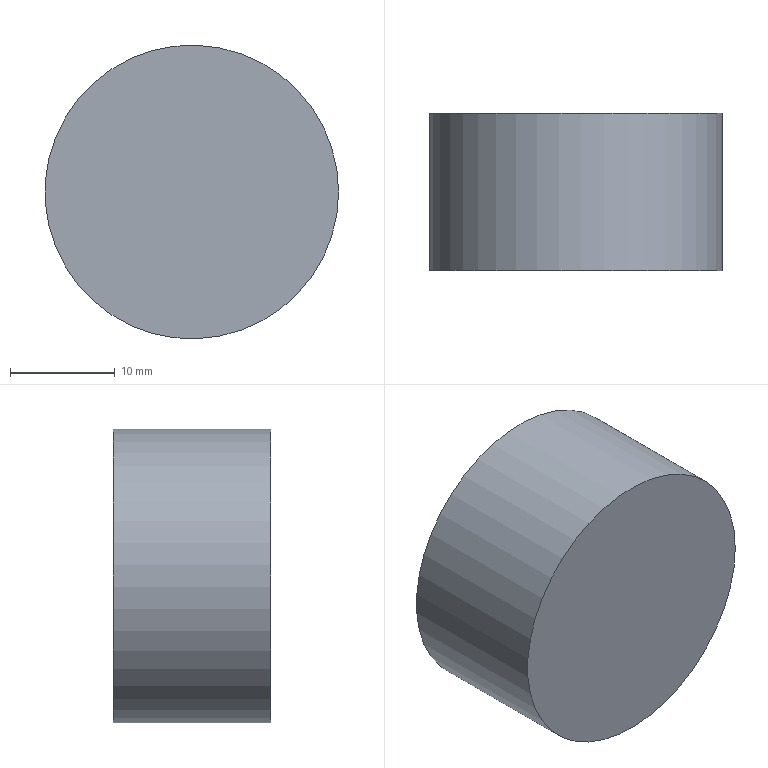Component | NX | CUP | 1 solid | 5 faces | box 28 x 15 x 28 mm | volume 5435 mm3 | plane 3 | cylinder 2 | commonest cylinder face diameters 28 x1 22 x1
STEP:
#1=CARTESIAN_POINT('',(0.,0.,0.));
#2=DIRECTION('',(0.,0.,1.));
#3=DIRECTION('',(1.,0.,0.));
#4=AXIS2_PLACEMENT_3D('',#1,#2,#3);
#5=CARTESIAN_POINT('',(14.,-47.923,-93.));
#6=VERTEX_POINT('',#5);
#7=CARTESIAN_POINT('',(0.,-47.923,-93.));
#8=DIRECTION('',(0.,1.,0.));
#9=DIRECTION('',(1.,0.,0.));
#10=AXIS2_PLACEMENT_3D('',#7,#8,#9);
#11=CIRCLE('',#10,14.);
#12=CARTESIAN_POINT('',(0.,-47.923,-93.));
#13=DIRECTION('',(0.,-1.,0.));
#14=DIRECTION('',(-1.,0.,0.));
#15=AXIS2_PLACEMENT_3D('',#12,#13,#14);
#16=CYLINDRICAL_SURFACE('',#15,14.);
#17=CARTESIAN_POINT('',(9.425,0.));
#18=DIRECTION('',(-1.,0.));
#19=VECTOR('',#18,1.);
#20=LINE('',#17,#19);
#21=(GEOMETRIC_REPRESENTATION_CONTEXT(2)PARAMETRIC_REPRESENTATION_CONTEXT()REPRESENTATION_CONTEXT('',''));
#22=DEFINITIONAL_REPRESENTATION('',(#20),#21);
#23=PCURVE('',#16,#22);
#24=CARTESIAN_POINT('',(0.,-47.923,-93.));
#25=DIRECTION('',(0.,1.,0.));
#26=DIRECTION('',(1.,0.,0.));
#27=AXIS2_PLACEMENT_3D('',#24,#25,#26);
#28=PLANE('',#27);
#29=CARTESIAN_POINT('',(0.,0.));
#30=DIRECTION('',(1.,0.));
#31=AXIS2_PLACEMENT_2D('',#29,#30);
#32=CIRCLE('',#31,14.);
#33=(GEOMETRIC_REPRESENTATION_CONTEXT(2)PARAMETRIC_REPRESENTATION_CONTEXT()REPRESENTATION_CONTEXT('',''));
#34=DEFINITIONAL_REPRESENTATION('',(#32),#33);
#35=PCURVE('',#28,#34);
#36=SURFACE_CURVE('',#11,(#23,#35),.PCURVE_S1.);
#37=EDGE_CURVE('',#6,#6,#36,.T.);
#38=ORIENTED_EDGE('',*,*,#37,.F.);
#39=CARTESIAN_POINT('',(14.,-62.923,-93.));
#40=VERTEX_POINT('',#39);
#41=CARTESIAN_POINT('',(14.,-47.923,-93.));
#42=CARTESIAN_POINT('',(14.,-62.923,-93.));
#43=B_SPLINE_CURVE_WITH_KNOTS('',1,(#41,#42),.UNSPECIFIED.,.F.,.F.,(2,2),(0.,15.),.PIECEWISE_BEZIER_KNOTS.);
#44=CARTESIAN_POINT('',(9.425,0.));
#45=DIRECTION('',(0.,1.));
#46=VECTOR('',#45,1.);
#47=LINE('',#44,#46);
#48=(GEOMETRIC_REPRESENTATION_CONTEXT(2)PARAMETRIC_REPRESENTATION_CONTEXT()REPRESENTATION_CONTEXT('',''));
#49=DEFINITIONAL_REPRESENTATION('',(#47),#48);
#50=PCURVE('',#16,#49);
#51=CARTESIAN_POINT('',(3.142,0.));
#52=DIRECTION('',(0.,1.));
#53=VECTOR('',#52,1.);
#54=LINE('',#51,#53);
#55=(GEOMETRIC_REPRESENTATION_CONTEXT(2)PARAMETRIC_REPRESENTATION_CONTEXT()REPRESENTATION_CONTEXT('',''));
#56=DEFINITIONAL_REPRESENTATION('',(#54),#55);
#57=PCURVE('',#16,#56);
#58=SEAM_CURVE('',#43,(#50,#57),.PCURVE_S1.);
#59=EDGE_CURVE('',#6,#40,#58,.T.);
#60=ORIENTED_EDGE('',*,*,#59,.T.);
#61=CARTESIAN_POINT('',(0.,-62.923,-93.));
#62=DIRECTION('',(0.,1.,0.));
#63=DIRECTION('',(1.,0.,0.));
#64=AXIS2_PLACEMENT_3D('',#61,#62,#63);
#65=CIRCLE('',#64,14.);
#66=CARTESIAN_POINT('',(9.425,15.));
#67=DIRECTION('',(-1.,0.));
#68=VECTOR('',#67,1.);
#69=LINE('',#66,#68);
#70=(GEOMETRIC_REPRESENTATION_CONTEXT(2)PARAMETRIC_REPRESENTATION_CONTEXT()REPRESENTATION_CONTEXT('',''));
#71=DEFINITIONAL_REPRESENTATION('',(#69),#70);
#72=PCURVE('',#16,#71);
#73=CARTESIAN_POINT('',(0.,-62.923,-93.));
#74=DIRECTION('',(0.,1.,0.));
#75=DIRECTION('',(1.,0.,0.));
#76=AXIS2_PLACEMENT_3D('',#73,#74,#75);
#77=PLANE('',#76);
#78=CARTESIAN_POINT('',(0.,0.));
#79=DIRECTION('',(1.,0.));
#80=AXIS2_PLACEMENT_2D('',#78,#79);
#81=CIRCLE('',#80,14.);
#82=(GEOMETRIC_REPRESENTATION_CONTEXT(2)PARAMETRIC_REPRESENTATION_CONTEXT()REPRESENTATION_CONTEXT('',''));
#83=DEFINITIONAL_REPRESENTATION('',(#81),#82);
#84=PCURVE('',#77,#83);
#85=SURFACE_CURVE('',#65,(#72,#84),.PCURVE_S1.);
#86=EDGE_CURVE('',#40,#40,#85,.T.);
#87=ORIENTED_EDGE('',*,*,#86,.T.);
#88=ORIENTED_EDGE('',*,*,#59,.F.);
#89=EDGE_LOOP('',(#38,#60,#87,#88));
#90=FACE_BOUND('',#89,.T.);
#91=ADVANCED_FACE('',(#90),#16,.T.);
#92=CARTESIAN_POINT('',(11.,-47.923,-93.));
#93=VERTEX_POINT('',#92);
#94=CARTESIAN_POINT('',(0.,-47.923,-93.));
#95=DIRECTION('',(0.,1.,0.));
#96=DIRECTION('',(1.,0.,0.));
#97=AXIS2_PLACEMENT_3D('',#94,#95,#96);
#98=CIRCLE('',#97,11.);
#99=CARTESIAN_POINT('',(0.,0.));
#100=DIRECTION('',(1.,0.));
#101=AXIS2_PLACEMENT_2D('',#99,#100);
#102=CIRCLE('',#101,11.);
#103=(GEOMETRIC_REPRESENTATION_CONTEXT(2)PARAMETRIC_REPRESENTATION_CONTEXT()REPRESENTATION_CONTEXT('',''));
#104=DEFINITIONAL_REPRESENTATION('',(#102),#103);
#105=PCURVE('',#28,#104);
#106=CARTESIAN_POINT('',(0.,-57.923,-93.));
#107=DIRECTION('',(0.,1.,0.));
#108=DIRECTION('',(1.,0.,0.));
#109=AXIS2_PLACEMENT_3D('',#106,#107,#108);
#110=CYLINDRICAL_SURFACE('',#109,11.);
#111=CARTESIAN_POINT('',(0.,10.));
#112=DIRECTION('',(1.,0.));
#113=VECTOR('',#112,1.);
#114=LINE('',#111,#113);
#115=(GEOMETRIC_REPRESENTATION_CONTEXT(2)PARAMETRIC_REPRESENTATION_CONTEXT()REPRESENTATION_CONTEXT('',''));
#116=DEFINITIONAL_REPRESENTATION('',(#114),#115);
#117=PCURVE('',#110,#116);
#118=SURFACE_CURVE('',#98,(#105,#117),.PCURVE_S1.);
#119=EDGE_CURVE('',#93,#93,#118,.T.);
#120=ORIENTED_EDGE('',*,*,#119,.F.);
#121=EDGE_LOOP('',(#120));
#122=FACE_BOUND('',#121,.T.);
#123=ORIENTED_EDGE('',*,*,#37,.T.);
#124=EDGE_LOOP('',(#123));
#125=FACE_BOUND('',#124,.T.);
#126=ADVANCED_FACE('',(#122,#125),#28,.T.);
#127=ORIENTED_EDGE('',*,*,#86,.F.);
#128=EDGE_LOOP('',(#127));
#129=FACE_BOUND('',#128,.T.);
#130=ADVANCED_FACE('',(#129),#77,.F.);
#131=CARTESIAN_POINT('',(11.,-57.923,-93.));
#132=VERTEX_POINT('',#131);
#133=CARTESIAN_POINT('',(0.,-57.923,-93.));
#134=DIRECTION('',(0.,-1.,0.));
#135=DIRECTION('',(1.,0.,0.));
#136=AXIS2_PLACEMENT_3D('',#133,#134,#135);
#137=CIRCLE('',#136,11.);
#138=CARTESIAN_POINT('',(6.283,0.));
#139=DIRECTION('',(-1.,0.));
#140=VECTOR('',#139,1.);
#141=LINE('',#138,#140);
#142=(GEOMETRIC_REPRESENTATION_CONTEXT(2)PARAMETRIC_REPRESENTATION_CONTEXT()REPRESENTATION_CONTEXT('',''));
#143=DEFINITIONAL_REPRESENTATION('',(#141),#142);
#144=PCURVE('',#110,#143);
#145=CARTESIAN_POINT('',(0.,-57.923,-93.));
#146=DIRECTION('',(0.,1.,0.));
#147=DIRECTION('',(1.,0.,0.));
#148=AXIS2_PLACEMENT_3D('',#145,#146,#147);
#149=PLANE('',#148);
#150=CARTESIAN_POINT('',(11.,0.));
#151=CARTESIAN_POINT('',(11.,-19.053));
#152=CARTESIAN_POINT('',(-5.5,-9.526));
#153=CARTESIAN_POINT('',(-22.,-0.));
#154=CARTESIAN_POINT('',(-5.5,9.526));
#155=CARTESIAN_POINT('',(11.,19.053));
#156=CARTESIAN_POINT('',(11.,0.));
#157=(BOUNDED_CURVE()B_SPLINE_CURVE(2,(#150,#151,#152,#153,#154,#155,#156),.UNSPECIFIED.,.T.,.F.)B_SPLINE_CURVE_WITH_KNOTS((1,2,2,2,2,1),(-2.094,0.,2.094,4.189,6.283,8.378),.UNSPECIFIED.)CURVE()GEOMETRIC_REPRESENTATION_ITEM()RATIONAL_B_SPLINE_CURVE((1.,0.5,1.,0.5,1.,0.5,1.))REPRESENTATION_ITEM(''));
#158=(GEOMETRIC_REPRESENTATION_CONTEXT(2)PARAMETRIC_REPRESENTATION_CONTEXT()REPRESENTATION_CONTEXT('',''));
#159=DEFINITIONAL_REPRESENTATION('',(#157),#158);
#160=PCURVE('',#149,#159);
#161=SURFACE_CURVE('',#137,(#144,#160),.PCURVE_S1.);
#162=EDGE_CURVE('',#132,#132,#161,.T.);
#163=ORIENTED_EDGE('',*,*,#162,.F.);
#164=CARTESIAN_POINT('',(11.,-57.923,-93.));
#165=CARTESIAN_POINT('',(11.,-47.923,-93.));
#166=B_SPLINE_CURVE_WITH_KNOTS('',1,(#164,#165),.UNSPECIFIED.,.F.,.F.,(2,2),(0.,10.),.PIECEWISE_BEZIER_KNOTS.);
#167=CARTESIAN_POINT('',(6.283,0.));
#168=DIRECTION('',(0.,1.));
#169=VECTOR('',#168,1.);
#170=LINE('',#167,#169);
#171=(GEOMETRIC_REPRESENTATION_CONTEXT(2)PARAMETRIC_REPRESENTATION_CONTEXT()REPRESENTATION_CONTEXT('',''));
#172=DEFINITIONAL_REPRESENTATION('',(#170),#171);
#173=PCURVE('',#110,#172);
#174=CARTESIAN_POINT('',(0.,0.));
#175=DIRECTION('',(0.,1.));
#176=VECTOR('',#175,1.);
#177=LINE('',#174,#176);
#178=(GEOMETRIC_REPRESENTATION_CONTEXT(2)PARAMETRIC_REPRESENTATION_CONTEXT()REPRESENTATION_CONTEXT('',''));
#179=DEFINITIONAL_REPRESENTATION('',(#177),#178);
#180=PCURVE('',#110,#179);
#181=SEAM_CURVE('',#166,(#173,#180),.PCURVE_S1.);
#182=EDGE_CURVE('',#132,#93,#181,.T.);
#183=ORIENTED_EDGE('',*,*,#182,.T.);
#184=ORIENTED_EDGE('',*,*,#119,.F.);
#185=ORIENTED_EDGE('',*,*,#182,.F.);
#186=EDGE_LOOP('',(#163,#183,#184,#185));
#187=FACE_BOUND('',#186,.F.);
#188=ADVANCED_FACE('',(#187),#110,.F.);
#189=ORIENTED_EDGE('',*,*,#162,.F.);
#190=EDGE_LOOP('',(#189));
#191=FACE_BOUND('',#190,.T.);
#192=ADVANCED_FACE('',(#191),#149,.T.);
#193=CLOSED_SHELL('',(#91,#126,#130,#188,#192));
#194=MANIFOLD_SOLID_BREP('',#193);
#195=(LENGTH_UNIT()NAMED_UNIT(*)SI_UNIT(.MILLI.,.METRE.));
#196=UNCERTAINTY_MEASURE_WITH_UNIT(LENGTH_MEASURE(0.00001),#195,'','');
#197=(NAMED_UNIT(*)PLANE_ANGLE_UNIT()SI_UNIT($,.RADIAN.));
#198=(NAMED_UNIT(*)SI_UNIT($,.STERADIAN.)SOLID_ANGLE_UNIT());
#199=(GEOMETRIC_REPRESENTATION_CONTEXT(3)GLOBAL_UNCERTAINTY_ASSIGNED_CONTEXT((#196))GLOBAL_UNIT_ASSIGNED_CONTEXT((#195,#197,#198))REPRESENTATION_CONTEXT('',''));
#200=ADVANCED_BREP_SHAPE_REPRESENTATION('',(#4,#194),#199);